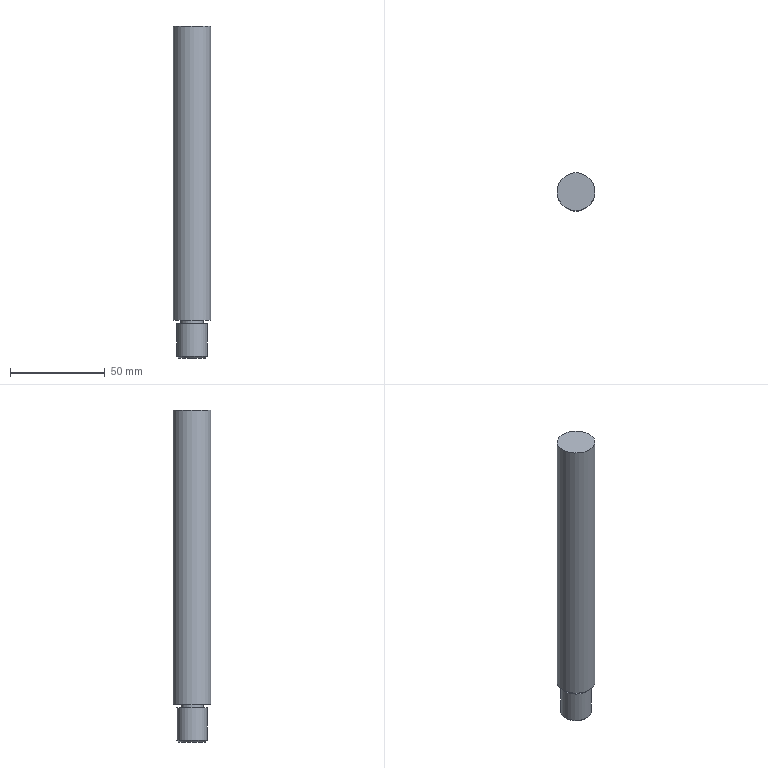Component | NX | CH3404_2-6 | 1 solid | 8 faces | box 20 x 20 x 175 mm | volume 52516 mm3 | plane 4 | cylinder 3 | cone 1 | commonest cylinder face diameters 20 x1 12 x1 16 x1
STEP:
#1=CARTESIAN_POINT('',(0.,0.,0.));
#2=DIRECTION('',(0.,0.,1.));
#3=DIRECTION('',(1.,0.,0.));
#4=AXIS2_PLACEMENT_3D('',#1,#2,#3);
#5=CARTESIAN_POINT('',(20.,-0.,-129.));
#6=VERTEX_POINT('',#5);
#7=CARTESIAN_POINT('',(30.,-0.,-129.));
#8=DIRECTION('',(0.,0.,-1.));
#9=DIRECTION('',(-1.,0.,0.));
#10=AXIS2_PLACEMENT_3D('',#7,#8,#9);
#11=CIRCLE('',#10,10.);
#12=CARTESIAN_POINT('',(30.,-0.,-149.));
#13=DIRECTION('',(0.,0.,-1.));
#14=DIRECTION('',(-1.,0.,0.));
#15=AXIS2_PLACEMENT_3D('',#12,#13,#14);
#16=CYLINDRICAL_SURFACE('',#15,10.);
#17=CARTESIAN_POINT('',(0.,-20.));
#18=DIRECTION('',(1.,0.));
#19=VECTOR('',#18,1.);
#20=LINE('',#17,#19);
#21=(GEOMETRIC_REPRESENTATION_CONTEXT(2)PARAMETRIC_REPRESENTATION_CONTEXT()REPRESENTATION_CONTEXT('',''));
#22=DEFINITIONAL_REPRESENTATION('',(#20),#21);
#23=PCURVE('',#16,#22);
#24=CARTESIAN_POINT('',(30.,-10.,-129.));
#25=DIRECTION('',(0.,0.,1.));
#26=DIRECTION('',(1.,0.,0.));
#27=AXIS2_PLACEMENT_3D('',#24,#25,#26);
#28=PLANE('',#27);
#29=CARTESIAN_POINT('',(-10.,10.));
#30=CARTESIAN_POINT('',(-10.,27.321));
#31=CARTESIAN_POINT('',(5.,18.66));
#32=CARTESIAN_POINT('',(20.,10.));
#33=CARTESIAN_POINT('',(5.,1.34));
#34=CARTESIAN_POINT('',(-10.,-7.321));
#35=CARTESIAN_POINT('',(-10.,10.));
#36=(BOUNDED_CURVE()B_SPLINE_CURVE(2,(#29,#30,#31,#32,#33,#34,#35),.UNSPECIFIED.,.T.,.F.)B_SPLINE_CURVE_WITH_KNOTS((1,2,2,2,2,1),(-2.094,0.,2.094,4.189,6.283,8.378),.UNSPECIFIED.)CURVE()GEOMETRIC_REPRESENTATION_ITEM()RATIONAL_B_SPLINE_CURVE((1.,0.5,1.,0.5,1.,0.5,1.))REPRESENTATION_ITEM(''));
#37=(GEOMETRIC_REPRESENTATION_CONTEXT(2)PARAMETRIC_REPRESENTATION_CONTEXT()REPRESENTATION_CONTEXT('',''));
#38=DEFINITIONAL_REPRESENTATION('',(#36),#37);
#39=PCURVE('',#28,#38);
#40=SURFACE_CURVE('',#11,(#23,#39),.PCURVE_S1.);
#41=EDGE_CURVE('',#6,#6,#40,.T.);
#42=ORIENTED_EDGE('',*,*,#41,.F.);
#43=CARTESIAN_POINT('',(20.,-0.,26.));
#44=VERTEX_POINT('',#43);
#45=CARTESIAN_POINT('',(20.,-0.,26.));
#46=CARTESIAN_POINT('',(20.,-0.,-129.));
#47=B_SPLINE_CURVE_WITH_KNOTS('',1,(#45,#46),.UNSPECIFIED.,.F.,.F.,(2,2),(-175.,-20.),.PIECEWISE_BEZIER_KNOTS.);
#48=CARTESIAN_POINT('',(0.,0.));
#49=DIRECTION('',(0.,1.));
#50=VECTOR('',#49,1.);
#51=LINE('',#48,#50);
#52=(GEOMETRIC_REPRESENTATION_CONTEXT(2)PARAMETRIC_REPRESENTATION_CONTEXT()REPRESENTATION_CONTEXT('',''));
#53=DEFINITIONAL_REPRESENTATION('',(#51),#52);
#54=PCURVE('',#16,#53);
#55=CARTESIAN_POINT('',(6.283,0.));
#56=DIRECTION('',(0.,1.));
#57=VECTOR('',#56,1.);
#58=LINE('',#55,#57);
#59=(GEOMETRIC_REPRESENTATION_CONTEXT(2)PARAMETRIC_REPRESENTATION_CONTEXT()REPRESENTATION_CONTEXT('',''));
#60=DEFINITIONAL_REPRESENTATION('',(#58),#59);
#61=PCURVE('',#16,#60);
#62=SEAM_CURVE('',#47,(#54,#61),.PCURVE_S1.);
#63=EDGE_CURVE('',#44,#6,#62,.T.);
#64=ORIENTED_EDGE('',*,*,#63,.F.);
#65=CARTESIAN_POINT('',(30.,-0.,26.));
#66=DIRECTION('',(0.,0.,-1.));
#67=DIRECTION('',(-1.,0.,0.));
#68=AXIS2_PLACEMENT_3D('',#65,#66,#67);
#69=CIRCLE('',#68,10.);
#70=CARTESIAN_POINT('',(0.,-175.));
#71=DIRECTION('',(1.,0.));
#72=VECTOR('',#71,1.);
#73=LINE('',#70,#72);
#74=(GEOMETRIC_REPRESENTATION_CONTEXT(2)PARAMETRIC_REPRESENTATION_CONTEXT()REPRESENTATION_CONTEXT('',''));
#75=DEFINITIONAL_REPRESENTATION('',(#73),#74);
#76=PCURVE('',#16,#75);
#77=CARTESIAN_POINT('',(30.,-0.,26.));
#78=DIRECTION('',(0.,0.,-1.));
#79=DIRECTION('',(-1.,0.,0.));
#80=AXIS2_PLACEMENT_3D('',#77,#78,#79);
#81=PLANE('',#80);
#82=CARTESIAN_POINT('',(0.,0.));
#83=DIRECTION('',(1.,0.));
#84=AXIS2_PLACEMENT_2D('',#82,#83);
#85=CIRCLE('',#84,10.);
#86=(GEOMETRIC_REPRESENTATION_CONTEXT(2)PARAMETRIC_REPRESENTATION_CONTEXT()REPRESENTATION_CONTEXT('',''));
#87=DEFINITIONAL_REPRESENTATION('',(#85),#86);
#88=PCURVE('',#81,#87);
#89=SURFACE_CURVE('',#69,(#76,#88),.PCURVE_S1.);
#90=EDGE_CURVE('',#44,#44,#89,.T.);
#91=ORIENTED_EDGE('',*,*,#90,.T.);
#92=ORIENTED_EDGE('',*,*,#63,.T.);
#93=EDGE_LOOP('',(#42,#64,#91,#92));
#94=FACE_BOUND('',#93,.T.);
#95=ADVANCED_FACE('',(#94),#16,.T.);
#96=CARTESIAN_POINT('',(24.,-0.,-129.));
#97=VERTEX_POINT('',#96);
#98=CARTESIAN_POINT('',(30.,-0.,-129.));
#99=DIRECTION('',(0.,0.,-1.));
#100=DIRECTION('',(-1.,0.,0.));
#101=AXIS2_PLACEMENT_3D('',#98,#99,#100);
#102=CIRCLE('',#101,6.);
#103=CARTESIAN_POINT('',(-6.,10.));
#104=CARTESIAN_POINT('',(-6.,20.392));
#105=CARTESIAN_POINT('',(3.,15.196));
#106=CARTESIAN_POINT('',(12.,10.));
#107=CARTESIAN_POINT('',(3.,4.804));
#108=CARTESIAN_POINT('',(-6.,-0.3923));
#109=CARTESIAN_POINT('',(-6.,10.));
#110=(BOUNDED_CURVE()B_SPLINE_CURVE(2,(#103,#104,#105,#106,#107,#108,#109),.UNSPECIFIED.,.T.,.F.)B_SPLINE_CURVE_WITH_KNOTS((1,2,2,2,2,1),(-2.094,0.,2.094,4.189,6.283,8.378),.UNSPECIFIED.)CURVE()GEOMETRIC_REPRESENTATION_ITEM()RATIONAL_B_SPLINE_CURVE((1.,0.5,1.,0.5,1.,0.5,1.))REPRESENTATION_ITEM(''));
#111=(GEOMETRIC_REPRESENTATION_CONTEXT(2)PARAMETRIC_REPRESENTATION_CONTEXT()REPRESENTATION_CONTEXT('',''));
#112=DEFINITIONAL_REPRESENTATION('',(#110),#111);
#113=PCURVE('',#28,#112);
#114=CARTESIAN_POINT('',(30.,-0.,-149.));
#115=DIRECTION('',(0.,0.,-1.));
#116=DIRECTION('',(-1.,0.,0.));
#117=AXIS2_PLACEMENT_3D('',#114,#115,#116);
#118=CYLINDRICAL_SURFACE('',#117,6.);
#119=CARTESIAN_POINT('',(0.,-20.));
#120=DIRECTION('',(1.,0.));
#121=VECTOR('',#120,1.);
#122=LINE('',#119,#121);
#123=(GEOMETRIC_REPRESENTATION_CONTEXT(2)PARAMETRIC_REPRESENTATION_CONTEXT()REPRESENTATION_CONTEXT('',''));
#124=DEFINITIONAL_REPRESENTATION('',(#122),#123);
#125=PCURVE('',#118,#124);
#126=SURFACE_CURVE('',#102,(#113,#125),.PCURVE_S1.);
#127=EDGE_CURVE('',#97,#97,#126,.T.);
#128=ORIENTED_EDGE('',*,*,#127,.F.);
#129=EDGE_LOOP('',(#128));
#130=FACE_BOUND('',#129,.T.);
#131=ORIENTED_EDGE('',*,*,#41,.T.);
#132=EDGE_LOOP('',(#131));
#133=FACE_BOUND('',#132,.T.);
#134=ADVANCED_FACE('',(#130,#133),#28,.F.);
#135=CARTESIAN_POINT('',(24.,-0.,-131.));
#136=VERTEX_POINT('',#135);
#137=CARTESIAN_POINT('',(30.,-0.,-131.));
#138=DIRECTION('',(0.,0.,-1.));
#139=DIRECTION('',(-1.,0.,0.));
#140=AXIS2_PLACEMENT_3D('',#137,#138,#139);
#141=CIRCLE('',#140,6.);
#142=CARTESIAN_POINT('',(0.,-18.));
#143=DIRECTION('',(1.,0.));
#144=VECTOR('',#143,1.);
#145=LINE('',#142,#144);
#146=(GEOMETRIC_REPRESENTATION_CONTEXT(2)PARAMETRIC_REPRESENTATION_CONTEXT()REPRESENTATION_CONTEXT('',''));
#147=DEFINITIONAL_REPRESENTATION('',(#145),#146);
#148=PCURVE('',#118,#147);
#149=CARTESIAN_POINT('',(30.,-6.,-131.));
#150=DIRECTION('',(0.,0.,-1.));
#151=DIRECTION('',(-1.,0.,0.));
#152=AXIS2_PLACEMENT_3D('',#149,#150,#151);
#153=PLANE('',#152);
#154=CARTESIAN_POINT('',(0.,6.));
#155=DIRECTION('',(1.,0.));
#156=AXIS2_PLACEMENT_2D('',#154,#155);
#157=CIRCLE('',#156,6.);
#158=(GEOMETRIC_REPRESENTATION_CONTEXT(2)PARAMETRIC_REPRESENTATION_CONTEXT()REPRESENTATION_CONTEXT('',''));
#159=DEFINITIONAL_REPRESENTATION('',(#157),#158);
#160=PCURVE('',#153,#159);
#161=SURFACE_CURVE('',#141,(#148,#160),.PCURVE_S1.);
#162=EDGE_CURVE('',#136,#136,#161,.T.);
#163=ORIENTED_EDGE('',*,*,#162,.F.);
#164=CARTESIAN_POINT('',(24.,-0.,-129.));
#165=CARTESIAN_POINT('',(24.,-0.,-131.));
#166=B_SPLINE_CURVE_WITH_KNOTS('',1,(#164,#165),.UNSPECIFIED.,.F.,.F.,(2,2),(-20.,-18.),.PIECEWISE_BEZIER_KNOTS.);
#167=CARTESIAN_POINT('',(0.,0.));
#168=DIRECTION('',(0.,1.));
#169=VECTOR('',#168,1.);
#170=LINE('',#167,#169);
#171=(GEOMETRIC_REPRESENTATION_CONTEXT(2)PARAMETRIC_REPRESENTATION_CONTEXT()REPRESENTATION_CONTEXT('',''));
#172=DEFINITIONAL_REPRESENTATION('',(#170),#171);
#173=PCURVE('',#118,#172);
#174=CARTESIAN_POINT('',(6.283,0.));
#175=DIRECTION('',(0.,1.));
#176=VECTOR('',#175,1.);
#177=LINE('',#174,#176);
#178=(GEOMETRIC_REPRESENTATION_CONTEXT(2)PARAMETRIC_REPRESENTATION_CONTEXT()REPRESENTATION_CONTEXT('',''));
#179=DEFINITIONAL_REPRESENTATION('',(#177),#178);
#180=PCURVE('',#118,#179);
#181=SEAM_CURVE('',#166,(#173,#180),.PCURVE_S1.);
#182=EDGE_CURVE('',#97,#136,#181,.T.);
#183=ORIENTED_EDGE('',*,*,#182,.F.);
#184=ORIENTED_EDGE('',*,*,#127,.T.);
#185=ORIENTED_EDGE('',*,*,#182,.T.);
#186=EDGE_LOOP('',(#163,#183,#184,#185));
#187=FACE_BOUND('',#186,.T.);
#188=ADVANCED_FACE('',(#187),#118,.T.);
#189=CARTESIAN_POINT('',(22.,-0.,-131.));
#190=VERTEX_POINT('',#189);
#191=CARTESIAN_POINT('',(30.,-0.,-131.));
#192=DIRECTION('',(0.,0.,-1.));
#193=DIRECTION('',(-1.,0.,0.));
#194=AXIS2_PLACEMENT_3D('',#191,#192,#193);
#195=CIRCLE('',#194,8.);
#196=CARTESIAN_POINT('',(0.,6.));
#197=DIRECTION('',(1.,0.));
#198=AXIS2_PLACEMENT_2D('',#196,#197);
#199=CIRCLE('',#198,8.);
#200=(GEOMETRIC_REPRESENTATION_CONTEXT(2)PARAMETRIC_REPRESENTATION_CONTEXT()REPRESENTATION_CONTEXT('',''));
#201=DEFINITIONAL_REPRESENTATION('',(#199),#200);
#202=PCURVE('',#153,#201);
#203=CARTESIAN_POINT('',(30.,-0.,-149.));
#204=DIRECTION('',(0.,0.,-1.));
#205=DIRECTION('',(-1.,0.,0.));
#206=AXIS2_PLACEMENT_3D('',#203,#204,#205);
#207=CYLINDRICAL_SURFACE('',#206,8.);
#208=CARTESIAN_POINT('',(0.,-18.));
#209=DIRECTION('',(1.,0.));
#210=VECTOR('',#209,1.);
#211=LINE('',#208,#210);
#212=(GEOMETRIC_REPRESENTATION_CONTEXT(2)PARAMETRIC_REPRESENTATION_CONTEXT()REPRESENTATION_CONTEXT('',''));
#213=DEFINITIONAL_REPRESENTATION('',(#211),#212);
#214=PCURVE('',#207,#213);
#215=SURFACE_CURVE('',#195,(#202,#214),.PCURVE_S1.);
#216=EDGE_CURVE('',#190,#190,#215,.T.);
#217=ORIENTED_EDGE('',*,*,#216,.F.);
#218=EDGE_LOOP('',(#217));
#219=FACE_BOUND('',#218,.T.);
#220=ORIENTED_EDGE('',*,*,#162,.T.);
#221=EDGE_LOOP('',(#220));
#222=FACE_BOUND('',#221,.T.);
#223=ADVANCED_FACE('',(#219,#222),#153,.F.);
#224=CARTESIAN_POINT('',(38.,-0.,-148.));
#225=VERTEX_POINT('',#224);
#226=CARTESIAN_POINT('',(22.,-0.,-148.));
#227=VERTEX_POINT('',#226);
#228=CARTESIAN_POINT('',(30.,-0.,-148.));
#229=DIRECTION('',(0.,0.,1.));
#230=DIRECTION('',(1.,0.,0.));
#231=AXIS2_PLACEMENT_3D('',#228,#229,#230);
#232=CIRCLE('',#231,8.);
#233=CARTESIAN_POINT('',(3.142,-1.));
#234=DIRECTION('',(-1.,0.));
#235=VECTOR('',#234,1.);
#236=LINE('',#233,#235);
#237=(GEOMETRIC_REPRESENTATION_CONTEXT(2)PARAMETRIC_REPRESENTATION_CONTEXT()REPRESENTATION_CONTEXT('',''));
#238=DEFINITIONAL_REPRESENTATION('',(#236),#237);
#239=PCURVE('',#207,#238);
#240=CARTESIAN_POINT('',(30.,-0.,-149.));
#241=DIRECTION('',(0.,0.,1.));
#242=DIRECTION('',(1.,0.,0.));
#243=AXIS2_PLACEMENT_3D('',#240,#241,#242);
#244=CONICAL_SURFACE('',#243,7.,0.7854);
#245=CARTESIAN_POINT('',(0.,1.));
#246=DIRECTION('',(1.,0.));
#247=VECTOR('',#246,1.);
#248=LINE('',#245,#247);
#249=(GEOMETRIC_REPRESENTATION_CONTEXT(2)PARAMETRIC_REPRESENTATION_CONTEXT()REPRESENTATION_CONTEXT('',''));
#250=DEFINITIONAL_REPRESENTATION('',(#248),#249);
#251=PCURVE('',#244,#250);
#252=SURFACE_CURVE('',#232,(#239,#251),.PCURVE_S1.);
#253=EDGE_CURVE('',#225,#227,#252,.T.);
#254=ORIENTED_EDGE('',*,*,#253,.T.);
#255=CARTESIAN_POINT('',(22.,-0.,-131.));
#256=CARTESIAN_POINT('',(22.,-0.,-148.));
#257=B_SPLINE_CURVE_WITH_KNOTS('',1,(#255,#256),.UNSPECIFIED.,.F.,.F.,(2,2),(-18.,-1.),.PIECEWISE_BEZIER_KNOTS.);
#258=CARTESIAN_POINT('',(0.,0.));
#259=DIRECTION('',(0.,1.));
#260=VECTOR('',#259,1.);
#261=LINE('',#258,#260);
#262=(GEOMETRIC_REPRESENTATION_CONTEXT(2)PARAMETRIC_REPRESENTATION_CONTEXT()REPRESENTATION_CONTEXT('',''));
#263=DEFINITIONAL_REPRESENTATION('',(#261),#262);
#264=PCURVE('',#207,#263);
#265=CARTESIAN_POINT('',(6.283,0.));
#266=DIRECTION('',(0.,1.));
#267=VECTOR('',#266,1.);
#268=LINE('',#265,#267);
#269=(GEOMETRIC_REPRESENTATION_CONTEXT(2)PARAMETRIC_REPRESENTATION_CONTEXT()REPRESENTATION_CONTEXT('',''));
#270=DEFINITIONAL_REPRESENTATION('',(#268),#269);
#271=PCURVE('',#207,#270);
#272=SEAM_CURVE('',#257,(#264,#271),.PCURVE_S1.);
#273=EDGE_CURVE('',#190,#227,#272,.T.);
#274=ORIENTED_EDGE('',*,*,#273,.F.);
#275=ORIENTED_EDGE('',*,*,#216,.T.);
#276=ORIENTED_EDGE('',*,*,#273,.T.);
#277=CARTESIAN_POINT('',(30.,-0.,-148.));
#278=DIRECTION('',(0.,0.,1.));
#279=DIRECTION('',(1.,0.,0.));
#280=AXIS2_PLACEMENT_3D('',#277,#278,#279);
#281=CIRCLE('',#280,8.);
#282=CARTESIAN_POINT('',(9.425,-1.));
#283=DIRECTION('',(-1.,0.));
#284=VECTOR('',#283,1.);
#285=LINE('',#282,#284);
#286=(GEOMETRIC_REPRESENTATION_CONTEXT(2)PARAMETRIC_REPRESENTATION_CONTEXT()REPRESENTATION_CONTEXT('',''));
#287=DEFINITIONAL_REPRESENTATION('',(#285),#286);
#288=PCURVE('',#207,#287);
#289=CARTESIAN_POINT('',(0.,1.));
#290=DIRECTION('',(1.,0.));
#291=VECTOR('',#290,1.);
#292=LINE('',#289,#291);
#293=(GEOMETRIC_REPRESENTATION_CONTEXT(2)PARAMETRIC_REPRESENTATION_CONTEXT()REPRESENTATION_CONTEXT('',''));
#294=DEFINITIONAL_REPRESENTATION('',(#292),#293);
#295=PCURVE('',#244,#294);
#296=SURFACE_CURVE('',#281,(#288,#295),.PCURVE_S1.);
#297=EDGE_CURVE('',#227,#225,#296,.T.);
#298=ORIENTED_EDGE('',*,*,#297,.T.);
#299=EDGE_LOOP('',(#254,#274,#275,#276,#298));
#300=FACE_BOUND('',#299,.T.);
#301=ADVANCED_FACE('',(#300),#207,.T.);
#302=CARTESIAN_POINT('',(37.,-0.,-149.));
#303=VERTEX_POINT('',#302);
#304=CARTESIAN_POINT('',(30.,-0.,-149.));
#305=DIRECTION('',(0.,0.,-1.));
#306=DIRECTION('',(1.,0.,0.));
#307=AXIS2_PLACEMENT_3D('',#304,#305,#306);
#308=CIRCLE('',#307,7.);
#309=CARTESIAN_POINT('',(30.,-8.,-149.));
#310=DIRECTION('',(0.,0.,1.));
#311=DIRECTION('',(1.,0.,0.));
#312=AXIS2_PLACEMENT_3D('',#309,#310,#311);
#313=PLANE('',#312);
#314=CARTESIAN_POINT('',(7.,8.));
#315=CARTESIAN_POINT('',(7.,-4.124));
#316=CARTESIAN_POINT('',(-3.5,1.938));
#317=CARTESIAN_POINT('',(-14.,8.));
#318=CARTESIAN_POINT('',(-3.5,14.062));
#319=CARTESIAN_POINT('',(7.,20.124));
#320=CARTESIAN_POINT('',(7.,8.));
#321=(BOUNDED_CURVE()B_SPLINE_CURVE(2,(#314,#315,#316,#317,#318,#319,#320),.UNSPECIFIED.,.T.,.F.)B_SPLINE_CURVE_WITH_KNOTS((1,2,2,2,2,1),(-2.094,0.,2.094,4.189,6.283,8.378),.UNSPECIFIED.)CURVE()GEOMETRIC_REPRESENTATION_ITEM()RATIONAL_B_SPLINE_CURVE((1.,0.5,1.,0.5,1.,0.5,1.))REPRESENTATION_ITEM(''));
#322=(GEOMETRIC_REPRESENTATION_CONTEXT(2)PARAMETRIC_REPRESENTATION_CONTEXT()REPRESENTATION_CONTEXT('',''));
#323=DEFINITIONAL_REPRESENTATION('',(#321),#322);
#324=PCURVE('',#313,#323);
#325=CARTESIAN_POINT('',(6.283,0.));
#326=DIRECTION('',(-1.,0.));
#327=VECTOR('',#326,1.);
#328=LINE('',#325,#327);
#329=(GEOMETRIC_REPRESENTATION_CONTEXT(2)PARAMETRIC_REPRESENTATION_CONTEXT()REPRESENTATION_CONTEXT('',''));
#330=DEFINITIONAL_REPRESENTATION('',(#328),#329);
#331=PCURVE('',#244,#330);
#332=SURFACE_CURVE('',#308,(#324,#331),.PCURVE_S1.);
#333=EDGE_CURVE('',#303,#303,#332,.T.);
#334=ORIENTED_EDGE('',*,*,#333,.T.);
#335=EDGE_LOOP('',(#334));
#336=FACE_BOUND('',#335,.T.);
#337=ADVANCED_FACE('',(#336),#313,.F.);
#338=ORIENTED_EDGE('',*,*,#90,.F.);
#339=EDGE_LOOP('',(#338));
#340=FACE_BOUND('',#339,.T.);
#341=ADVANCED_FACE('',(#340),#81,.F.);
#342=ORIENTED_EDGE('',*,*,#253,.F.);
#343=CARTESIAN_POINT('',(37.,-0.,-149.));
#344=CARTESIAN_POINT('',(38.,-0.,-148.));
#345=B_SPLINE_CURVE_WITH_KNOTS('',1,(#343,#344),.UNSPECIFIED.,.F.,.F.,(2,2),(0.,1.414),.PIECEWISE_BEZIER_KNOTS.);
#346=CARTESIAN_POINT('',(0.,0.));
#347=DIRECTION('',(0.,1.));
#348=VECTOR('',#347,1.);
#349=LINE('',#346,#348);
#350=(GEOMETRIC_REPRESENTATION_CONTEXT(2)PARAMETRIC_REPRESENTATION_CONTEXT()REPRESENTATION_CONTEXT('',''));
#351=DEFINITIONAL_REPRESENTATION('',(#349),#350);
#352=PCURVE('',#244,#351);
#353=CARTESIAN_POINT('',(6.283,0.));
#354=DIRECTION('',(0.,1.));
#355=VECTOR('',#354,1.);
#356=LINE('',#353,#355);
#357=(GEOMETRIC_REPRESENTATION_CONTEXT(2)PARAMETRIC_REPRESENTATION_CONTEXT()REPRESENTATION_CONTEXT('',''));
#358=DEFINITIONAL_REPRESENTATION('',(#356),#357);
#359=PCURVE('',#244,#358);
#360=SEAM_CURVE('',#345,(#352,#359),.PCURVE_S1.);
#361=EDGE_CURVE('',#303,#225,#360,.T.);
#362=ORIENTED_EDGE('',*,*,#361,.F.);
#363=ORIENTED_EDGE('',*,*,#333,.F.);
#364=ORIENTED_EDGE('',*,*,#361,.T.);
#365=ORIENTED_EDGE('',*,*,#297,.F.);
#366=EDGE_LOOP('',(#342,#362,#363,#364,#365));
#367=FACE_BOUND('',#366,.T.);
#368=ADVANCED_FACE('',(#367),#244,.T.);
#369=CLOSED_SHELL('',(#95,#134,#188,#223,#301,#337,#341,#368));
#370=MANIFOLD_SOLID_BREP('',#369);
#371=(LENGTH_UNIT()NAMED_UNIT(*)SI_UNIT(.MILLI.,.METRE.));
#372=UNCERTAINTY_MEASURE_WITH_UNIT(LENGTH_MEASURE(0.00001),#371,'','');
#373=(NAMED_UNIT(*)PLANE_ANGLE_UNIT()SI_UNIT($,.RADIAN.));
#374=(NAMED_UNIT(*)SI_UNIT($,.STERADIAN.)SOLID_ANGLE_UNIT());
#375=(GEOMETRIC_REPRESENTATION_CONTEXT(3)GLOBAL_UNCERTAINTY_ASSIGNED_CONTEXT((#372))GLOBAL_UNIT_ASSIGNED_CONTEXT((#371,#373,#374))REPRESENTATION_CONTEXT('',''));
#376=ADVANCED_BREP_SHAPE_REPRESENTATION('',(#4,#370),#375);